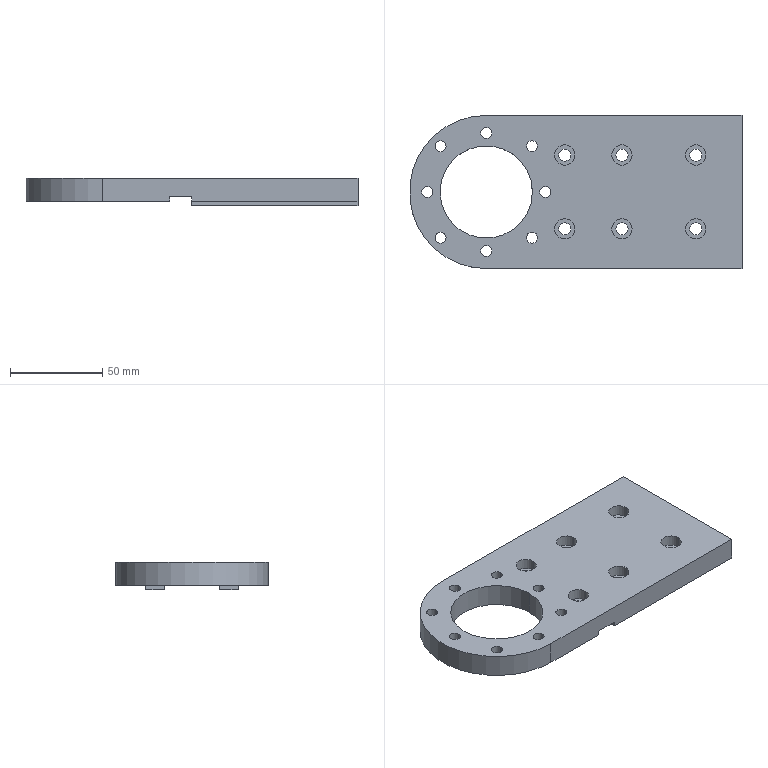Component | SolidWorks | Q1-A12-S21-Q1A.SLDASQ-1_Q1-A12-S21-Q1A-01A-2 | 1 solid | 66 faces | box 180 x 83 x 15 mm | volume 147213 mm3 | cylinder 43 | plane 23 | commonest cylinder face diameters 6 x16 11 x12 6.6 x12 50.01 x2 83 x1 | material S-45C
build123d program:
from build123d import *

# Parameters (mm, degrees)
SKETCH1_W                                            = 180
SKETCH1_H                                            = 83
BOSS_EXTRUDE1_DEPTH                                  = 15
SKETCH2_W                                            = 2.5
SKETCH2_H                                            = 16.5
SKETCH2_H_2                                          = 30
CUT_EXTRUDE1_DEPTH                                   = 186.33
CUT_EXTRUDE2_DEPTH                                   = 101.236
SKETCH4_W                                            = 12
SKETCH4_H                                            = 5
CUT_EXTRUDE3_DEPTH                                   = 124.345
F_25_5_25_5_DIAMETER_HOLE3_D                         = 50.01
SKETCH7_W                                            = 78
SKETCH7_H                                            = 2.5
CUT_EXTRUDE4_DEPTH                                   = 124.345
CYLINDRICAL_COUNTERSUNK_HOLE_FOR_M6_SOCK_D           = 6.6
CYLINDRICAL_COUNTERSUNK_HOLE_FOR_M6_SOCK_CBORE_D     = 11
CYLINDRICAL_COUNTERSUNK_HOLE_FOR_M6_SOCK_CBORE_DEPTH = 6
M6X1_0_TAPPED_HOLE1_D                                = 6


with BuildPart() as part:
    # Sketch1 → Boss-Extrude1 (new body)
    with BuildSketch(Plane.XY):
        Rectangle(SKETCH1_W, SKETCH1_H)
    extrude(amount=BOSS_EXTRUDE1_DEPTH)

    # Sketch2 → Cut-Extrude1 (cut, through all)
    with BuildSketch(Plane(origin=(90, 0, 0), x_dir=(0, 0, -1), z_dir=(1, 0, 0))):
        with Locations((-1.25, 33.25)):
            Rectangle(SKETCH2_W, SKETCH2_H)
        with Locations((-1.25, 0)):
            Rectangle(SKETCH2_W, SKETCH2_H_2)
        with Locations((-1.25, -33.25)):
            Rectangle(SKETCH2_W, SKETCH2_H)
    extrude(amount=-CUT_EXTRUDE1_DEPTH, mode=Mode.SUBTRACT)

    # Sketch3 → Cut-Extrude2 (cut, through all)
    with BuildSketch(Plane.XY.offset(15)):
        with BuildLine():
            ThreePointArc((-90, 0), (-77.845, 29.345), (-48.5, 41.5))
            Line((-48.5, 41.5), (-90, 41.5))
            Line((-90, 41.5), (-90, 0))
        make_face()
        with BuildLine():
            ThreePointArc((-48.5, -41.5), (-77.845, -29.345), (-90, 0))
            Line((-90, 0), (-90, -41.5))
            Line((-90, -41.5), (-48.5, -41.5))
        make_face()
    extrude(amount=-CUT_EXTRUDE2_DEPTH, mode=Mode.SUBTRACT)

    # Sketch4 → Cut-Extrude3 (cut, through all)
    with BuildSketch(Plane(origin=(0, 41.5, 0), x_dir=(1, 0, 0), z_dir=(0, 1, 0))):
        with Locations((-6, -2.5)):
            Rectangle(SKETCH4_W, SKETCH4_H)
    extrude(amount=-CUT_EXTRUDE3_DEPTH, mode=Mode.SUBTRACT)

    # 25.5 _25.5_ Diameter Hole3 (through all)
    with Locations(Plane.XY.offset(15)):
        with Locations((-48.5, 0)):
            Hole(F_25_5_25_5_DIAMETER_HOLE3_D / 2)

    # Sketch7 → Cut-Extrude4 (cut, through all)
    with BuildSketch(Plane(origin=(0, 41.5, 0), x_dir=(1, 0, 0), z_dir=(0, 1, 0))):
        with Locations((-51, -1.25)):
            Rectangle(SKETCH7_W, SKETCH7_H)
    extrude(amount=-CUT_EXTRUDE4_DEPTH, mode=Mode.SUBTRACT)

    # Cylindrical Countersunk Hole for M6 Sock (through all)
    with Locations(Plane.XY.offset(15)):
        with Locations((-6, 20), (-6, -20), (65, 20), (25, 20), (65, -20), (25, -20)):
            CounterBoreHole(CYLINDRICAL_COUNTERSUNK_HOLE_FOR_M6_SOCK_D / 2, CYLINDRICAL_COUNTERSUNK_HOLE_FOR_M6_SOCK_CBORE_D / 2, CYLINDRICAL_COUNTERSUNK_HOLE_FOR_M6_SOCK_CBORE_DEPTH)

    # M6x1.0 Tapped Hole1 (through all)
    with Locations(Plane.XY.offset(15)):
        with Locations((-16.5, 0), (-48.5, 32), (-80.5, 0), (-48.5, -32), (-73.249, 24.749), (-23.751, -24.749), (-23.751, 24.749), (-73.249, -24.749)):
            Hole(M6X1_0_TAPPED_HOLE1_D / 2)


solid = part.part

# Placed as in the assembly
solid = solid.moved(Location((48.5, 0, 147.5), (0, 0, 0)))